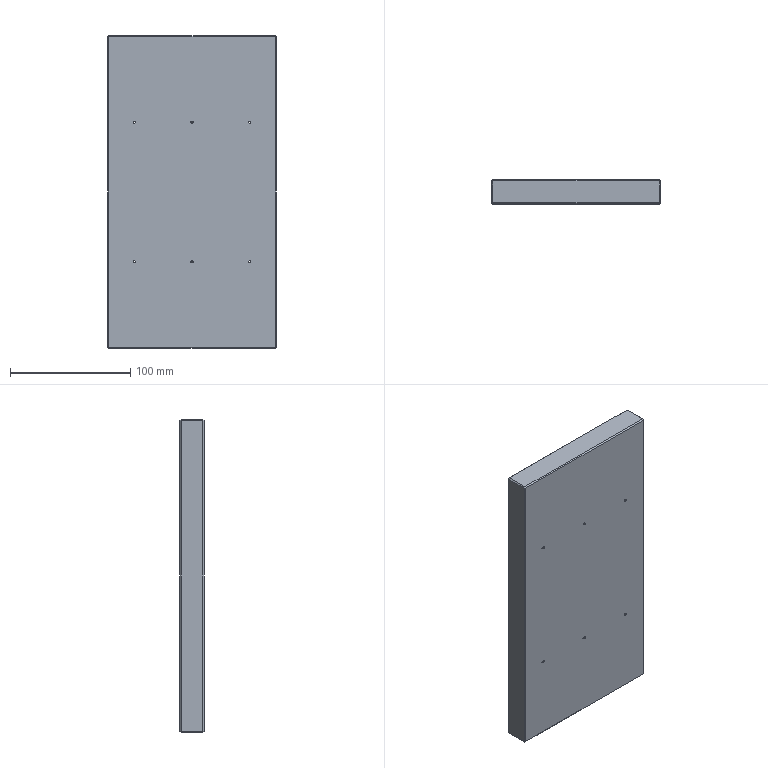Component | SolidWorks | UpperDieConnectingPlate1-1 | 1 solid | 50 faces | box 140 x 20 x 260 mm | volume 720750 mm3 | plane 26 | cylinder 12 | cone 12 | commonest cylinder face diameters 8.5 x12
build123d program:
from build123d import *

# Parameters (mm, degrees)
SKETCH1_W              = 140
SKETCH1_H              = 260
BOSS_EXTRUDE1_DEPTH    = 20
M10_TAPPED_HOLE1_D     = 8.5
M10_TAPPED_HOLE1_DEPTH = 18
M10_TAPPED_HOLE1_TIP   = 2.554
CHAMFER1_SIZE          = 1


with BuildPart() as part:
    # Sketch1 → Boss-Extrude1 (new body)
    with BuildSketch(Plane.XY):
        with Locations((70, 130)):
            Rectangle(SKETCH1_W, SKETCH1_H)
    extrude(amount=BOSS_EXTRUDE1_DEPTH)

    # M10 Tapped Hole1
    with Locations(Plane.XY.offset(20)):
        with Locations((22, 188), (70, 188), (118, 188), (118, 72), (70, 72), (22, 72)):
            Hole(M10_TAPPED_HOLE1_D / 2, depth=M10_TAPPED_HOLE1_DEPTH)
            with Locations((0, 0, -(M10_TAPPED_HOLE1_DEPTH + M10_TAPPED_HOLE1_TIP / 2))):  # 118° drill point
                Cone(0, M10_TAPPED_HOLE1_D / 2, M10_TAPPED_HOLE1_TIP, mode=Mode.SUBTRACT)

    # Chamfer1
    chamfer1_edges = [part.edges().sort_by_distance(p)[0] for p in [
        (140, 130, 20),
        (70, 260, 20),
        (0, 130, 20),
        (70, 260, 0),
        (140, 130, 0),
        (70, 0, 0),
        (0, 130, 0),
        (70, 0, 20),
        (0, 260, 10),
        (140, 260, 10),
        (140, 0, 10),
        (0, 0, 10),
    ]]
    chamfer(chamfer1_edges, length=CHAMFER1_SIZE)


solid = part.part

# Placed as in the assembly
solid = solid.moved(Location((-247.951, 623.269, 135), (-90, 0, 0)))